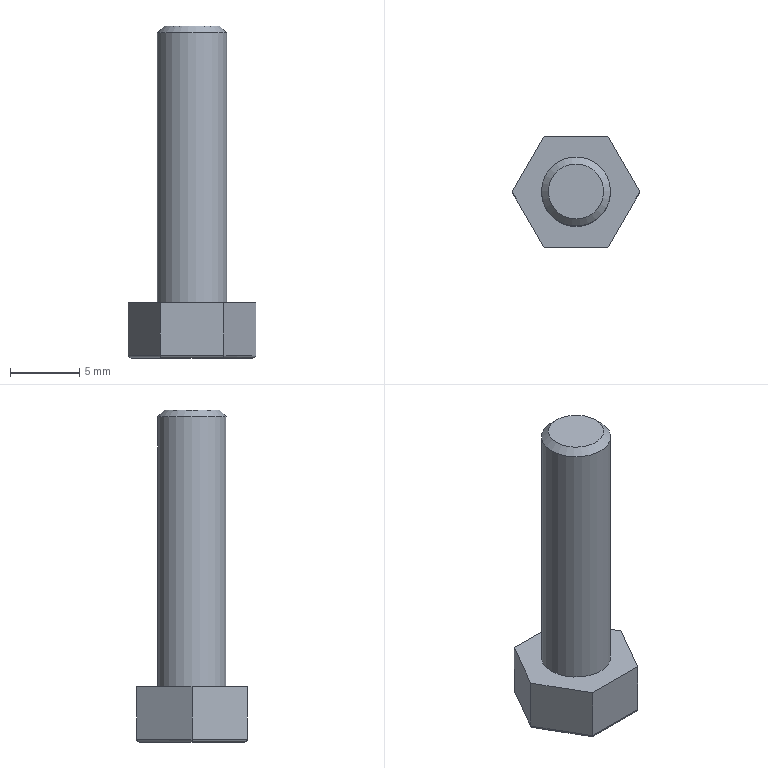Component | NX | BOLT_4 | 1 solid | 17 faces | box 9.24 x 8 x 24 mm | volume 612 mm3 | plane 9 | cylinder 7 | cone 1 | commonest cylinder face diameters 0.4 x6 5 x1
STEP:
#1=CARTESIAN_POINT('',(0.,0.,0.));
#2=DIRECTION('',(0.,0.,1.));
#3=DIRECTION('',(1.,0.,0.));
#4=AXIS2_PLACEMENT_3D('',#1,#2,#3);
#5=CARTESIAN_POINT('',(22.453,0.,12.));
#6=VERTEX_POINT('',#5);
#7=CARTESIAN_POINT('',(20.453,0.,12.));
#8=DIRECTION('',(0.,0.,1.));
#9=DIRECTION('',(1.,0.,0.));
#10=AXIS2_PLACEMENT_3D('',#7,#8,#9);
#11=CIRCLE('',#10,2.);
#12=CARTESIAN_POINT('',(20.453,0.,12.));
#13=DIRECTION('',(0.,0.,1.));
#14=DIRECTION('',(1.,0.,0.));
#15=AXIS2_PLACEMENT_3D('',#12,#13,#14);
#16=PLANE('',#15);
#17=CARTESIAN_POINT('',(0.,0.));
#18=DIRECTION('',(1.,0.));
#19=AXIS2_PLACEMENT_2D('',#17,#18);
#20=CIRCLE('',#19,2.);
#21=(GEOMETRIC_REPRESENTATION_CONTEXT(2)PARAMETRIC_REPRESENTATION_CONTEXT()REPRESENTATION_CONTEXT('',''));
#22=DEFINITIONAL_REPRESENTATION('',(#20),#21);
#23=PCURVE('',#16,#22);
#24=CARTESIAN_POINT('',(20.453,0.,11.5));
#25=DIRECTION('',(0.,0.,-1.));
#26=DIRECTION('',(-1.,0.,0.));
#27=AXIS2_PLACEMENT_3D('',#24,#25,#26);
#28=CONICAL_SURFACE('',#27,2.5,0.7854);
#29=CARTESIAN_POINT('',(9.425,-0.5));
#30=DIRECTION('',(-1.,0.));
#31=VECTOR('',#30,1.);
#32=LINE('',#29,#31);
#33=(GEOMETRIC_REPRESENTATION_CONTEXT(2)PARAMETRIC_REPRESENTATION_CONTEXT()REPRESENTATION_CONTEXT('',''));
#34=DEFINITIONAL_REPRESENTATION('',(#32),#33);
#35=PCURVE('',#28,#34);
#36=SURFACE_CURVE('',#11,(#23,#35),.PCURVE_S1.);
#37=EDGE_CURVE('',#6,#6,#36,.T.);
#38=ORIENTED_EDGE('',*,*,#37,.T.);
#39=EDGE_LOOP('',(#38));
#40=FACE_BOUND('',#39,.T.);
#41=ADVANCED_FACE('',(#40),#16,.T.);
#42=CARTESIAN_POINT('',(22.953,0.,11.5));
#43=VERTEX_POINT('',#42);
#44=CARTESIAN_POINT('',(17.953,-0.,11.5));
#45=VERTEX_POINT('',#44);
#46=CARTESIAN_POINT('',(20.453,0.,11.5));
#47=DIRECTION('',(0.,0.,-1.));
#48=DIRECTION('',(1.,0.,0.));
#49=AXIS2_PLACEMENT_3D('',#46,#47,#48);
#50=CIRCLE('',#49,2.5);
#51=CARTESIAN_POINT('',(20.453,0.,12.));
#52=DIRECTION('',(0.,0.,-1.));
#53=DIRECTION('',(-1.,0.,0.));
#54=AXIS2_PLACEMENT_3D('',#51,#52,#53);
#55=CYLINDRICAL_SURFACE('',#54,2.5);
#56=CARTESIAN_POINT('',(3.142,0.5));
#57=DIRECTION('',(1.,0.));
#58=VECTOR('',#57,1.);
#59=LINE('',#56,#58);
#60=(GEOMETRIC_REPRESENTATION_CONTEXT(2)PARAMETRIC_REPRESENTATION_CONTEXT()REPRESENTATION_CONTEXT('',''));
#61=DEFINITIONAL_REPRESENTATION('',(#59),#60);
#62=PCURVE('',#55,#61);
#63=CARTESIAN_POINT('',(3.142,0.));
#64=DIRECTION('',(1.,0.));
#65=VECTOR('',#64,1.);
#66=LINE('',#63,#65);
#67=(GEOMETRIC_REPRESENTATION_CONTEXT(2)PARAMETRIC_REPRESENTATION_CONTEXT()REPRESENTATION_CONTEXT('',''));
#68=DEFINITIONAL_REPRESENTATION('',(#66),#67);
#69=PCURVE('',#28,#68);
#70=SURFACE_CURVE('',#50,(#62,#69),.PCURVE_S1.);
#71=EDGE_CURVE('',#43,#45,#70,.T.);
#72=ORIENTED_EDGE('',*,*,#71,.T.);
#73=CARTESIAN_POINT('',(17.953,0.,-8.));
#74=VERTEX_POINT('',#73);
#75=CARTESIAN_POINT('',(17.953,0.,11.5));
#76=CARTESIAN_POINT('',(17.953,0.,-8.));
#77=B_SPLINE_CURVE_WITH_KNOTS('',1,(#75,#76),.UNSPECIFIED.,.F.,.F.,(2,2),(0.5,20.),.PIECEWISE_BEZIER_KNOTS.);
#78=CARTESIAN_POINT('',(6.283,0.));
#79=DIRECTION('',(0.,1.));
#80=VECTOR('',#79,1.);
#81=LINE('',#78,#80);
#82=(GEOMETRIC_REPRESENTATION_CONTEXT(2)PARAMETRIC_REPRESENTATION_CONTEXT()REPRESENTATION_CONTEXT('',''));
#83=DEFINITIONAL_REPRESENTATION('',(#81),#82);
#84=PCURVE('',#55,#83);
#85=CARTESIAN_POINT('',(0.,0.));
#86=DIRECTION('',(0.,1.));
#87=VECTOR('',#86,1.);
#88=LINE('',#85,#87);
#89=(GEOMETRIC_REPRESENTATION_CONTEXT(2)PARAMETRIC_REPRESENTATION_CONTEXT()REPRESENTATION_CONTEXT('',''));
#90=DEFINITIONAL_REPRESENTATION('',(#88),#89);
#91=PCURVE('',#55,#90);
#92=SEAM_CURVE('',#77,(#84,#91),.PCURVE_S1.);
#93=EDGE_CURVE('',#45,#74,#92,.T.);
#94=ORIENTED_EDGE('',*,*,#93,.T.);
#95=CARTESIAN_POINT('',(20.453,0.,-8.));
#96=DIRECTION('',(0.,0.,1.));
#97=DIRECTION('',(-1.,0.,0.));
#98=AXIS2_PLACEMENT_3D('',#95,#96,#97);
#99=CIRCLE('',#98,2.5);
#100=CARTESIAN_POINT('',(6.283,20.));
#101=DIRECTION('',(-1.,0.));
#102=VECTOR('',#101,1.);
#103=LINE('',#100,#102);
#104=(GEOMETRIC_REPRESENTATION_CONTEXT(2)PARAMETRIC_REPRESENTATION_CONTEXT()REPRESENTATION_CONTEXT('',''));
#105=DEFINITIONAL_REPRESENTATION('',(#103),#104);
#106=PCURVE('',#55,#105);
#107=CARTESIAN_POINT('',(20.453,0.,-8.));
#108=DIRECTION('',(0.,0.,-1.));
#109=DIRECTION('',(-1.,0.,0.));
#110=AXIS2_PLACEMENT_3D('',#107,#108,#109);
#111=PLANE('',#110);
#112=CARTESIAN_POINT('',(2.5,0.));
#113=CARTESIAN_POINT('',(2.5,-4.33));
#114=CARTESIAN_POINT('',(-1.25,-2.165));
#115=CARTESIAN_POINT('',(-5.,-0.));
#116=CARTESIAN_POINT('',(-1.25,2.165));
#117=CARTESIAN_POINT('',(2.5,4.33));
#118=CARTESIAN_POINT('',(2.5,0.));
#119=(BOUNDED_CURVE()B_SPLINE_CURVE(2,(#112,#113,#114,#115,#116,#117,#118),.UNSPECIFIED.,.T.,.F.)B_SPLINE_CURVE_WITH_KNOTS((1,2,2,2,2,1),(-2.094,0.,2.094,4.189,6.283,8.378),.UNSPECIFIED.)CURVE()GEOMETRIC_REPRESENTATION_ITEM()RATIONAL_B_SPLINE_CURVE((1.,0.5,1.,0.5,1.,0.5,1.))REPRESENTATION_ITEM(''));
#120=(GEOMETRIC_REPRESENTATION_CONTEXT(2)PARAMETRIC_REPRESENTATION_CONTEXT()REPRESENTATION_CONTEXT('',''));
#121=DEFINITIONAL_REPRESENTATION('',(#119),#120);
#122=PCURVE('',#111,#121);
#123=SURFACE_CURVE('',#99,(#106,#122),.PCURVE_S1.);
#124=EDGE_CURVE('',#74,#74,#123,.T.);
#125=ORIENTED_EDGE('',*,*,#124,.T.);
#126=ORIENTED_EDGE('',*,*,#93,.F.);
#127=CARTESIAN_POINT('',(20.453,0.,11.5));
#128=DIRECTION('',(0.,0.,-1.));
#129=DIRECTION('',(1.,0.,0.));
#130=AXIS2_PLACEMENT_3D('',#127,#128,#129);
#131=CIRCLE('',#130,2.5);
#132=CARTESIAN_POINT('',(-3.142,0.5));
#133=DIRECTION('',(1.,0.));
#134=VECTOR('',#133,1.);
#135=LINE('',#132,#134);
#136=(GEOMETRIC_REPRESENTATION_CONTEXT(2)PARAMETRIC_REPRESENTATION_CONTEXT()REPRESENTATION_CONTEXT('',''));
#137=DEFINITIONAL_REPRESENTATION('',(#135),#136);
#138=PCURVE('',#55,#137);
#139=CARTESIAN_POINT('',(3.142,0.));
#140=DIRECTION('',(1.,0.));
#141=VECTOR('',#140,1.);
#142=LINE('',#139,#141);
#143=(GEOMETRIC_REPRESENTATION_CONTEXT(2)PARAMETRIC_REPRESENTATION_CONTEXT()REPRESENTATION_CONTEXT('',''));
#144=DEFINITIONAL_REPRESENTATION('',(#142),#143);
#145=PCURVE('',#28,#144);
#146=SURFACE_CURVE('',#131,(#138,#145),.PCURVE_S1.);
#147=EDGE_CURVE('',#45,#43,#146,.T.);
#148=ORIENTED_EDGE('',*,*,#147,.T.);
#149=EDGE_LOOP('',(#72,#94,#125,#126,#148));
#150=FACE_BOUND('',#149,.T.);
#151=ADVANCED_FACE('',(#150),#55,.T.);
#152=CARTESIAN_POINT('',(18.143,4.,-11.8));
#153=VERTEX_POINT('',#152);
#154=CARTESIAN_POINT('',(18.143,4.,-8.));
#155=VERTEX_POINT('',#154);
#156=CARTESIAN_POINT('',(18.143,4.,-12.));
#157=DIRECTION('',(0.,0.,1.));
#158=VECTOR('',#157,1.);
#159=LINE('',#156,#158);
#160=CARTESIAN_POINT('',(15.834,-0.,-12.));
#161=DIRECTION('',(0.866,-0.5,0.));
#162=DIRECTION('',(-0.5,-0.866,0.));
#163=AXIS2_PLACEMENT_3D('',#160,#161,#162);
#164=PLANE('',#163);
#165=CARTESIAN_POINT('',(-4.619,0.));
#166=DIRECTION('',(0.,-1.));
#167=VECTOR('',#166,1.);
#168=LINE('',#165,#167);
#169=(GEOMETRIC_REPRESENTATION_CONTEXT(2)PARAMETRIC_REPRESENTATION_CONTEXT()REPRESENTATION_CONTEXT('',''));
#170=DEFINITIONAL_REPRESENTATION('',(#168),#169);
#171=PCURVE('',#164,#170);
#172=CARTESIAN_POINT('',(18.143,4.,-12.));
#173=DIRECTION('',(0.,-1.,0.));
#174=DIRECTION('',(0.,0.,1.));
#175=AXIS2_PLACEMENT_3D('',#172,#173,#174);
#176=PLANE('',#175);
#177=CARTESIAN_POINT('',(0.,0.));
#178=DIRECTION('',(1.,0.));
#179=VECTOR('',#178,1.);
#180=LINE('',#177,#179);
#181=(GEOMETRIC_REPRESENTATION_CONTEXT(2)PARAMETRIC_REPRESENTATION_CONTEXT()REPRESENTATION_CONTEXT('',''));
#182=DEFINITIONAL_REPRESENTATION('',(#180),#181);
#183=PCURVE('',#176,#182);
#184=SURFACE_CURVE('',#159,(#171,#183),.PCURVE_S1.);
#185=EDGE_CURVE('',#153,#155,#184,.T.);
#186=ORIENTED_EDGE('',*,*,#185,.F.);
#187=CARTESIAN_POINT('',(15.834,-0.,-11.8));
#188=VERTEX_POINT('',#187);
#189=CARTESIAN_POINT('',(15.834,-0.,-11.8));
#190=DIRECTION('',(-0.5,-0.866,0.));
#191=VECTOR('',#190,1.);
#192=LINE('',#189,#191);
#193=CARTESIAN_POINT('',(0.,-0.2));
#194=DIRECTION('',(1.,0.));
#195=VECTOR('',#194,1.);
#196=LINE('',#193,#195);
#197=(GEOMETRIC_REPRESENTATION_CONTEXT(2)PARAMETRIC_REPRESENTATION_CONTEXT()REPRESENTATION_CONTEXT('',''));
#198=DEFINITIONAL_REPRESENTATION('',(#196),#197);
#199=PCURVE('',#164,#198);
#200=CARTESIAN_POINT('',(17.162,1.9,-11.8));
#201=DIRECTION('',(-0.5,-0.866,0.));
#202=DIRECTION('',(-0.866,0.5,0.));
#203=AXIS2_PLACEMENT_3D('',#200,#201,#202);
#204=CYLINDRICAL_SURFACE('',#203,0.2);
#205=CARTESIAN_POINT('',(0.,2.309));
#206=DIRECTION('',(0.,1.));
#207=VECTOR('',#206,1.);
#208=LINE('',#205,#207);
#209=(GEOMETRIC_REPRESENTATION_CONTEXT(2)PARAMETRIC_REPRESENTATION_CONTEXT()REPRESENTATION_CONTEXT('',''));
#210=DEFINITIONAL_REPRESENTATION('',(#208),#209);
#211=PCURVE('',#204,#210);
#212=SURFACE_CURVE('',#192,(#199,#211),.PCURVE_S1.);
#213=EDGE_CURVE('',#153,#188,#212,.T.);
#214=ORIENTED_EDGE('',*,*,#213,.T.);
#215=CARTESIAN_POINT('',(15.834,-0.,-8.));
#216=VERTEX_POINT('',#215);
#217=CARTESIAN_POINT('',(15.834,-0.,-12.));
#218=DIRECTION('',(0.,0.,1.));
#219=VECTOR('',#218,1.);
#220=LINE('',#217,#219);
#221=CARTESIAN_POINT('',(0.,0.));
#222=DIRECTION('',(0.,-1.));
#223=VECTOR('',#222,1.);
#224=LINE('',#221,#223);
#225=(GEOMETRIC_REPRESENTATION_CONTEXT(2)PARAMETRIC_REPRESENTATION_CONTEXT()REPRESENTATION_CONTEXT('',''));
#226=DEFINITIONAL_REPRESENTATION('',(#224),#225);
#227=PCURVE('',#164,#226);
#228=CARTESIAN_POINT('',(18.143,-4.,-12.));
#229=DIRECTION('',(0.866,0.5,0.));
#230=DIRECTION('',(0.5,-0.866,0.));
#231=AXIS2_PLACEMENT_3D('',#228,#229,#230);
#232=PLANE('',#231);
#233=CARTESIAN_POINT('',(-4.619,0.));
#234=DIRECTION('',(0.,-1.));
#235=VECTOR('',#234,1.);
#236=LINE('',#233,#235);
#237=(GEOMETRIC_REPRESENTATION_CONTEXT(2)PARAMETRIC_REPRESENTATION_CONTEXT()REPRESENTATION_CONTEXT('',''));
#238=DEFINITIONAL_REPRESENTATION('',(#236),#237);
#239=PCURVE('',#232,#238);
#240=SURFACE_CURVE('',#220,(#227,#239),.PCURVE_S1.);
#241=EDGE_CURVE('',#188,#216,#240,.T.);
#242=ORIENTED_EDGE('',*,*,#241,.T.);
#243=CARTESIAN_POINT('',(15.834,-0.,-8.));
#244=DIRECTION('',(0.5,0.866,0.));
#245=VECTOR('',#244,1.);
#246=LINE('',#243,#245);
#247=CARTESIAN_POINT('',(0.,-4.));
#248=DIRECTION('',(-1.,0.));
#249=VECTOR('',#248,1.);
#250=LINE('',#247,#249);
#251=(GEOMETRIC_REPRESENTATION_CONTEXT(2)PARAMETRIC_REPRESENTATION_CONTEXT()REPRESENTATION_CONTEXT('',''));
#252=DEFINITIONAL_REPRESENTATION('',(#250),#251);
#253=PCURVE('',#164,#252);
#254=CARTESIAN_POINT('',(4.619,-0.));
#255=DIRECTION('',(-0.5,0.866));
#256=VECTOR('',#255,1.);
#257=LINE('',#254,#256);
#258=(GEOMETRIC_REPRESENTATION_CONTEXT(2)PARAMETRIC_REPRESENTATION_CONTEXT()REPRESENTATION_CONTEXT('',''));
#259=DEFINITIONAL_REPRESENTATION('',(#257),#258);
#260=PCURVE('',#111,#259);
#261=SURFACE_CURVE('',#246,(#253,#260),.PCURVE_S1.);
#262=EDGE_CURVE('',#216,#155,#261,.T.);
#263=ORIENTED_EDGE('',*,*,#262,.T.);
#264=EDGE_LOOP('',(#186,#214,#242,#263));
#265=FACE_BOUND('',#264,.T.);
#266=ADVANCED_FACE('',(#265),#164,.F.);
#267=CARTESIAN_POINT('',(22.762,4.,-11.8));
#268=VERTEX_POINT('',#267);
#269=CARTESIAN_POINT('',(22.762,4.,-8.));
#270=VERTEX_POINT('',#269);
#271=CARTESIAN_POINT('',(22.762,4.,-12.));
#272=DIRECTION('',(0.,0.,1.));
#273=VECTOR('',#272,1.);
#274=LINE('',#271,#273);
#275=CARTESIAN_POINT('',(0.,-4.619));
#276=DIRECTION('',(1.,0.));
#277=VECTOR('',#276,1.);
#278=LINE('',#275,#277);
#279=(GEOMETRIC_REPRESENTATION_CONTEXT(2)PARAMETRIC_REPRESENTATION_CONTEXT()REPRESENTATION_CONTEXT('',''));
#280=DEFINITIONAL_REPRESENTATION('',(#278),#279);
#281=PCURVE('',#176,#280);
#282=CARTESIAN_POINT('',(22.762,4.,-12.));
#283=DIRECTION('',(-0.866,-0.5,0.));
#284=DIRECTION('',(-0.5,0.866,0.));
#285=AXIS2_PLACEMENT_3D('',#282,#283,#284);
#286=PLANE('',#285);
#287=CARTESIAN_POINT('',(0.,0.));
#288=DIRECTION('',(0.,-1.));
#289=VECTOR('',#288,1.);
#290=LINE('',#287,#289);
#291=(GEOMETRIC_REPRESENTATION_CONTEXT(2)PARAMETRIC_REPRESENTATION_CONTEXT()REPRESENTATION_CONTEXT('',''));
#292=DEFINITIONAL_REPRESENTATION('',(#290),#291);
#293=PCURVE('',#286,#292);
#294=SURFACE_CURVE('',#274,(#281,#293),.PCURVE_S1.);
#295=EDGE_CURVE('',#268,#270,#294,.T.);
#296=ORIENTED_EDGE('',*,*,#295,.F.);
#297=CARTESIAN_POINT('',(18.143,4.,-11.8));
#298=DIRECTION('',(-1.,0.,0.));
#299=VECTOR('',#298,1.);
#300=LINE('',#297,#299);
#301=CARTESIAN_POINT('',(0.2,0.));
#302=DIRECTION('',(0.,1.));
#303=VECTOR('',#302,1.);
#304=LINE('',#301,#303);
#305=(GEOMETRIC_REPRESENTATION_CONTEXT(2)PARAMETRIC_REPRESENTATION_CONTEXT()REPRESENTATION_CONTEXT('',''));
#306=DEFINITIONAL_REPRESENTATION('',(#304),#305);
#307=PCURVE('',#176,#306);
#308=CARTESIAN_POINT('',(20.453,3.8,-11.8));
#309=DIRECTION('',(-1.,0.,0.));
#310=DIRECTION('',(0.,0.,1.));
#311=AXIS2_PLACEMENT_3D('',#308,#309,#310);
#312=CYLINDRICAL_SURFACE('',#311,0.2);
#313=CARTESIAN_POINT('',(1.571,2.309));
#314=DIRECTION('',(0.,1.));
#315=VECTOR('',#314,1.);
#316=LINE('',#313,#315);
#317=(GEOMETRIC_REPRESENTATION_CONTEXT(2)PARAMETRIC_REPRESENTATION_CONTEXT()REPRESENTATION_CONTEXT('',''));
#318=DEFINITIONAL_REPRESENTATION('',(#316),#317);
#319=PCURVE('',#312,#318);
#320=SURFACE_CURVE('',#300,(#307,#319),.PCURVE_S1.);
#321=EDGE_CURVE('',#268,#153,#320,.T.);
#322=ORIENTED_EDGE('',*,*,#321,.T.);
#323=ORIENTED_EDGE('',*,*,#185,.T.);
#324=CARTESIAN_POINT('',(18.143,4.,-8.));
#325=DIRECTION('',(1.,0.,0.));
#326=VECTOR('',#325,1.);
#327=LINE('',#324,#326);
#328=CARTESIAN_POINT('',(4.,0.));
#329=DIRECTION('',(0.,-1.));
#330=VECTOR('',#329,1.);
#331=LINE('',#328,#330);
#332=(GEOMETRIC_REPRESENTATION_CONTEXT(2)PARAMETRIC_REPRESENTATION_CONTEXT()REPRESENTATION_CONTEXT('',''));
#333=DEFINITIONAL_REPRESENTATION('',(#331),#332);
#334=PCURVE('',#176,#333);
#335=CARTESIAN_POINT('',(2.309,4.));
#336=DIRECTION('',(-1.,0.));
#337=VECTOR('',#336,1.);
#338=LINE('',#335,#337);
#339=(GEOMETRIC_REPRESENTATION_CONTEXT(2)PARAMETRIC_REPRESENTATION_CONTEXT()REPRESENTATION_CONTEXT('',''));
#340=DEFINITIONAL_REPRESENTATION('',(#338),#339);
#341=PCURVE('',#111,#340);
#342=SURFACE_CURVE('',#327,(#334,#341),.PCURVE_S1.);
#343=EDGE_CURVE('',#155,#270,#342,.T.);
#344=ORIENTED_EDGE('',*,*,#343,.T.);
#345=EDGE_LOOP('',(#296,#322,#323,#344));
#346=FACE_BOUND('',#345,.T.);
#347=ADVANCED_FACE('',(#346),#176,.F.);
#348=CARTESIAN_POINT('',(25.072,0.,-11.8));
#349=VERTEX_POINT('',#348);
#350=CARTESIAN_POINT('',(25.072,0.,-8.));
#351=VERTEX_POINT('',#350);
#352=CARTESIAN_POINT('',(25.072,0.,-12.));
#353=DIRECTION('',(0.,0.,1.));
#354=VECTOR('',#353,1.);
#355=LINE('',#352,#354);
#356=CARTESIAN_POINT('',(-4.619,0.));
#357=DIRECTION('',(0.,-1.));
#358=VECTOR('',#357,1.);
#359=LINE('',#356,#358);
#360=(GEOMETRIC_REPRESENTATION_CONTEXT(2)PARAMETRIC_REPRESENTATION_CONTEXT()REPRESENTATION_CONTEXT('',''));
#361=DEFINITIONAL_REPRESENTATION('',(#359),#360);
#362=PCURVE('',#286,#361);
#363=CARTESIAN_POINT('',(25.072,0.,-12.));
#364=DIRECTION('',(-0.866,0.5,0.));
#365=DIRECTION('',(0.5,0.866,0.));
#366=AXIS2_PLACEMENT_3D('',#363,#364,#365);
#367=PLANE('',#366);
#368=CARTESIAN_POINT('',(0.,0.));
#369=DIRECTION('',(0.,-1.));
#370=VECTOR('',#369,1.);
#371=LINE('',#368,#370);
#372=(GEOMETRIC_REPRESENTATION_CONTEXT(2)PARAMETRIC_REPRESENTATION_CONTEXT()REPRESENTATION_CONTEXT('',''));
#373=DEFINITIONAL_REPRESENTATION('',(#371),#372);
#374=PCURVE('',#367,#373);
#375=SURFACE_CURVE('',#355,(#362,#374),.PCURVE_S1.);
#376=EDGE_CURVE('',#349,#351,#375,.T.);
#377=ORIENTED_EDGE('',*,*,#376,.F.);
#378=CARTESIAN_POINT('',(22.762,4.,-11.8));
#379=DIRECTION('',(-0.5,0.866,0.));
#380=VECTOR('',#379,1.);
#381=LINE('',#378,#380);
#382=CARTESIAN_POINT('',(0.,-0.2));
#383=DIRECTION('',(1.,0.));
#384=VECTOR('',#383,1.);
#385=LINE('',#382,#384);
#386=(GEOMETRIC_REPRESENTATION_CONTEXT(2)PARAMETRIC_REPRESENTATION_CONTEXT()REPRESENTATION_CONTEXT('',''));
#387=DEFINITIONAL_REPRESENTATION('',(#385),#386);
#388=PCURVE('',#286,#387);
#389=CARTESIAN_POINT('',(23.744,1.9,-11.8));
#390=DIRECTION('',(-0.5,0.866,0.));
#391=DIRECTION('',(0.866,0.5,0.));
#392=AXIS2_PLACEMENT_3D('',#389,#390,#391);
#393=CYLINDRICAL_SURFACE('',#392,0.2);
#394=CARTESIAN_POINT('',(0.,2.309));
#395=DIRECTION('',(0.,1.));
#396=VECTOR('',#395,1.);
#397=LINE('',#394,#396);
#398=(GEOMETRIC_REPRESENTATION_CONTEXT(2)PARAMETRIC_REPRESENTATION_CONTEXT()REPRESENTATION_CONTEXT('',''));
#399=DEFINITIONAL_REPRESENTATION('',(#397),#398);
#400=PCURVE('',#393,#399);
#401=SURFACE_CURVE('',#381,(#388,#400),.PCURVE_S1.);
#402=EDGE_CURVE('',#349,#268,#401,.T.);
#403=ORIENTED_EDGE('',*,*,#402,.T.);
#404=ORIENTED_EDGE('',*,*,#295,.T.);
#405=CARTESIAN_POINT('',(22.762,4.,-8.));
#406=DIRECTION('',(0.5,-0.866,0.));
#407=VECTOR('',#406,1.);
#408=LINE('',#405,#407);
#409=CARTESIAN_POINT('',(0.,-4.));
#410=DIRECTION('',(-1.,0.));
#411=VECTOR('',#410,1.);
#412=LINE('',#409,#411);
#413=(GEOMETRIC_REPRESENTATION_CONTEXT(2)PARAMETRIC_REPRESENTATION_CONTEXT()REPRESENTATION_CONTEXT('',''));
#414=DEFINITIONAL_REPRESENTATION('',(#412),#413);
#415=PCURVE('',#286,#414);
#416=CARTESIAN_POINT('',(-2.309,4.));
#417=DIRECTION('',(-0.5,-0.866));
#418=VECTOR('',#417,1.);
#419=LINE('',#416,#418);
#420=(GEOMETRIC_REPRESENTATION_CONTEXT(2)PARAMETRIC_REPRESENTATION_CONTEXT()REPRESENTATION_CONTEXT('',''));
#421=DEFINITIONAL_REPRESENTATION('',(#419),#420);
#422=PCURVE('',#111,#421);
#423=SURFACE_CURVE('',#408,(#415,#422),.PCURVE_S1.);
#424=EDGE_CURVE('',#270,#351,#423,.T.);
#425=ORIENTED_EDGE('',*,*,#424,.T.);
#426=EDGE_LOOP('',(#377,#403,#404,#425));
#427=FACE_BOUND('',#426,.T.);
#428=ADVANCED_FACE('',(#427),#286,.F.);
#429=CARTESIAN_POINT('',(22.762,-4.,-11.8));
#430=VERTEX_POINT('',#429);
#431=CARTESIAN_POINT('',(22.762,-4.,-8.));
#432=VERTEX_POINT('',#431);
#433=CARTESIAN_POINT('',(22.762,-4.,-12.));
#434=DIRECTION('',(0.,0.,1.));
#435=VECTOR('',#434,1.);
#436=LINE('',#433,#435);
#437=CARTESIAN_POINT('',(-4.619,0.));
#438=DIRECTION('',(0.,-1.));
#439=VECTOR('',#438,1.);
#440=LINE('',#437,#439);
#441=(GEOMETRIC_REPRESENTATION_CONTEXT(2)PARAMETRIC_REPRESENTATION_CONTEXT()REPRESENTATION_CONTEXT('',''));
#442=DEFINITIONAL_REPRESENTATION('',(#440),#441);
#443=PCURVE('',#367,#442);
#444=CARTESIAN_POINT('',(22.762,-4.,-12.));
#445=DIRECTION('',(0.,1.,0.));
#446=DIRECTION('',(0.,0.,-1.));
#447=AXIS2_PLACEMENT_3D('',#444,#445,#446);
#448=PLANE('',#447);
#449=CARTESIAN_POINT('',(0.,0.));
#450=DIRECTION('',(-1.,0.));
#451=VECTOR('',#450,1.);
#452=LINE('',#449,#451);
#453=(GEOMETRIC_REPRESENTATION_CONTEXT(2)PARAMETRIC_REPRESENTATION_CONTEXT()REPRESENTATION_CONTEXT('',''));
#454=DEFINITIONAL_REPRESENTATION('',(#452),#453);
#455=PCURVE('',#448,#454);
#456=SURFACE_CURVE('',#436,(#443,#455),.PCURVE_S1.);
#457=EDGE_CURVE('',#430,#432,#456,.T.);
#458=ORIENTED_EDGE('',*,*,#457,.F.);
#459=CARTESIAN_POINT('',(25.072,0.,-11.8));
#460=DIRECTION('',(0.5,0.866,0.));
#461=VECTOR('',#460,1.);
#462=LINE('',#459,#461);
#463=CARTESIAN_POINT('',(0.,-0.2));
#464=DIRECTION('',(1.,0.));
#465=VECTOR('',#464,1.);
#466=LINE('',#463,#465);
#467=(GEOMETRIC_REPRESENTATION_CONTEXT(2)PARAMETRIC_REPRESENTATION_CONTEXT()REPRESENTATION_CONTEXT('',''));
#468=DEFINITIONAL_REPRESENTATION('',(#466),#467);
#469=PCURVE('',#367,#468);
#470=CARTESIAN_POINT('',(23.744,-1.9,-11.8));
#471=DIRECTION('',(0.5,0.866,0.));
#472=DIRECTION('',(0.866,-0.5,0.));
#473=AXIS2_PLACEMENT_3D('',#470,#471,#472);
#474=CYLINDRICAL_SURFACE('',#473,0.2);
#475=CARTESIAN_POINT('',(0.,2.309));
#476=DIRECTION('',(0.,1.));
#477=VECTOR('',#476,1.);
#478=LINE('',#475,#477);
#479=(GEOMETRIC_REPRESENTATION_CONTEXT(2)PARAMETRIC_REPRESENTATION_CONTEXT()REPRESENTATION_CONTEXT('',''));
#480=DEFINITIONAL_REPRESENTATION('',(#478),#479);
#481=PCURVE('',#474,#480);
#482=SURFACE_CURVE('',#462,(#469,#481),.PCURVE_S1.);
#483=EDGE_CURVE('',#430,#349,#482,.T.);
#484=ORIENTED_EDGE('',*,*,#483,.T.);
#485=ORIENTED_EDGE('',*,*,#376,.T.);
#486=CARTESIAN_POINT('',(25.072,0.,-8.));
#487=DIRECTION('',(-0.5,-0.866,0.));
#488=VECTOR('',#487,1.);
#489=LINE('',#486,#488);
#490=CARTESIAN_POINT('',(0.,-4.));
#491=DIRECTION('',(-1.,0.));
#492=VECTOR('',#491,1.);
#493=LINE('',#490,#492);
#494=(GEOMETRIC_REPRESENTATION_CONTEXT(2)PARAMETRIC_REPRESENTATION_CONTEXT()REPRESENTATION_CONTEXT('',''));
#495=DEFINITIONAL_REPRESENTATION('',(#493),#494);
#496=PCURVE('',#367,#495);
#497=CARTESIAN_POINT('',(-4.619,0.));
#498=DIRECTION('',(0.5,-0.866));
#499=VECTOR('',#498,1.);
#500=LINE('',#497,#499);
#501=(GEOMETRIC_REPRESENTATION_CONTEXT(2)PARAMETRIC_REPRESENTATION_CONTEXT()REPRESENTATION_CONTEXT('',''));
#502=DEFINITIONAL_REPRESENTATION('',(#500),#501);
#503=PCURVE('',#111,#502);
#504=SURFACE_CURVE('',#489,(#496,#503),.PCURVE_S1.);
#505=EDGE_CURVE('',#351,#432,#504,.T.);
#506=ORIENTED_EDGE('',*,*,#505,.T.);
#507=EDGE_LOOP('',(#458,#484,#485,#506));
#508=FACE_BOUND('',#507,.T.);
#509=ADVANCED_FACE('',(#508),#367,.F.);
#510=CARTESIAN_POINT('',(18.143,-4.,-11.8));
#511=VERTEX_POINT('',#510);
#512=CARTESIAN_POINT('',(18.143,-4.,-8.));
#513=VERTEX_POINT('',#512);
#514=CARTESIAN_POINT('',(18.143,-4.,-12.));
#515=DIRECTION('',(0.,0.,1.));
#516=VECTOR('',#515,1.);
#517=LINE('',#514,#516);
#518=CARTESIAN_POINT('',(0.,4.619));
#519=DIRECTION('',(-1.,0.));
#520=VECTOR('',#519,1.);
#521=LINE('',#518,#520);
#522=(GEOMETRIC_REPRESENTATION_CONTEXT(2)PARAMETRIC_REPRESENTATION_CONTEXT()REPRESENTATION_CONTEXT('',''));
#523=DEFINITIONAL_REPRESENTATION('',(#521),#522);
#524=PCURVE('',#448,#523);
#525=CARTESIAN_POINT('',(0.,0.));
#526=DIRECTION('',(0.,-1.));
#527=VECTOR('',#526,1.);
#528=LINE('',#525,#527);
#529=(GEOMETRIC_REPRESENTATION_CONTEXT(2)PARAMETRIC_REPRESENTATION_CONTEXT()REPRESENTATION_CONTEXT('',''));
#530=DEFINITIONAL_REPRESENTATION('',(#528),#529);
#531=PCURVE('',#232,#530);
#532=SURFACE_CURVE('',#517,(#524,#531),.PCURVE_S1.);
#533=EDGE_CURVE('',#511,#513,#532,.T.);
#534=ORIENTED_EDGE('',*,*,#533,.F.);
#535=CARTESIAN_POINT('',(22.762,-4.,-11.8));
#536=DIRECTION('',(1.,0.,0.));
#537=VECTOR('',#536,1.);
#538=LINE('',#535,#537);
#539=CARTESIAN_POINT('',(-0.2,0.));
#540=DIRECTION('',(0.,-1.));
#541=VECTOR('',#540,1.);
#542=LINE('',#539,#541);
#543=(GEOMETRIC_REPRESENTATION_CONTEXT(2)PARAMETRIC_REPRESENTATION_CONTEXT()REPRESENTATION_CONTEXT('',''));
#544=DEFINITIONAL_REPRESENTATION('',(#542),#543);
#545=PCURVE('',#448,#544);
#546=CARTESIAN_POINT('',(20.453,-3.8,-11.8));
#547=DIRECTION('',(1.,0.,0.));
#548=DIRECTION('',(0.,0.,-1.));
#549=AXIS2_PLACEMENT_3D('',#546,#547,#548);
#550=CYLINDRICAL_SURFACE('',#549,0.2);
#551=CARTESIAN_POINT('',(4.712,2.309));
#552=DIRECTION('',(0.,1.));
#553=VECTOR('',#552,1.);
#554=LINE('',#551,#553);
#555=(GEOMETRIC_REPRESENTATION_CONTEXT(2)PARAMETRIC_REPRESENTATION_CONTEXT()REPRESENTATION_CONTEXT('',''));
#556=DEFINITIONAL_REPRESENTATION('',(#554),#555);
#557=PCURVE('',#550,#556);
#558=SURFACE_CURVE('',#538,(#545,#557),.PCURVE_S1.);
#559=EDGE_CURVE('',#511,#430,#558,.T.);
#560=ORIENTED_EDGE('',*,*,#559,.T.);
#561=ORIENTED_EDGE('',*,*,#457,.T.);
#562=CARTESIAN_POINT('',(22.762,-4.,-8.));
#563=DIRECTION('',(-1.,0.,0.));
#564=VECTOR('',#563,1.);
#565=LINE('',#562,#564);
#566=CARTESIAN_POINT('',(-4.,0.));
#567=DIRECTION('',(0.,1.));
#568=VECTOR('',#567,1.);
#569=LINE('',#566,#568);
#570=(GEOMETRIC_REPRESENTATION_CONTEXT(2)PARAMETRIC_REPRESENTATION_CONTEXT()REPRESENTATION_CONTEXT('',''));
#571=DEFINITIONAL_REPRESENTATION('',(#569),#570);
#572=PCURVE('',#448,#571);
#573=CARTESIAN_POINT('',(-2.309,-4.));
#574=DIRECTION('',(1.,0.));
#575=VECTOR('',#574,1.);
#576=LINE('',#573,#575);
#577=(GEOMETRIC_REPRESENTATION_CONTEXT(2)PARAMETRIC_REPRESENTATION_CONTEXT()REPRESENTATION_CONTEXT('',''));
#578=DEFINITIONAL_REPRESENTATION('',(#576),#577);
#579=PCURVE('',#111,#578);
#580=SURFACE_CURVE('',#565,(#572,#579),.PCURVE_S1.);
#581=EDGE_CURVE('',#432,#513,#580,.T.);
#582=ORIENTED_EDGE('',*,*,#581,.T.);
#583=EDGE_LOOP('',(#534,#560,#561,#582));
#584=FACE_BOUND('',#583,.T.);
#585=ADVANCED_FACE('',(#584),#448,.F.);
#586=ORIENTED_EDGE('',*,*,#241,.F.);
#587=CARTESIAN_POINT('',(18.143,-4.,-11.8));
#588=DIRECTION('',(0.5,-0.866,0.));
#589=VECTOR('',#588,1.);
#590=LINE('',#587,#589);
#591=CARTESIAN_POINT('',(0.,-0.2));
#592=DIRECTION('',(1.,0.));
#593=VECTOR('',#592,1.);
#594=LINE('',#591,#593);
#595=(GEOMETRIC_REPRESENTATION_CONTEXT(2)PARAMETRIC_REPRESENTATION_CONTEXT()REPRESENTATION_CONTEXT('',''));
#596=DEFINITIONAL_REPRESENTATION('',(#594),#595);
#597=PCURVE('',#232,#596);
#598=CARTESIAN_POINT('',(17.162,-1.9,-11.8));
#599=DIRECTION('',(0.5,-0.866,0.));
#600=DIRECTION('',(-0.866,-0.5,0.));
#601=AXIS2_PLACEMENT_3D('',#598,#599,#600);
#602=CYLINDRICAL_SURFACE('',#601,0.2);
#603=CARTESIAN_POINT('',(0.,2.309));
#604=DIRECTION('',(0.,1.));
#605=VECTOR('',#604,1.);
#606=LINE('',#603,#605);
#607=(GEOMETRIC_REPRESENTATION_CONTEXT(2)PARAMETRIC_REPRESENTATION_CONTEXT()REPRESENTATION_CONTEXT('',''));
#608=DEFINITIONAL_REPRESENTATION('',(#606),#607);
#609=PCURVE('',#602,#608);
#610=SURFACE_CURVE('',#590,(#597,#609),.PCURVE_S1.);
#611=EDGE_CURVE('',#188,#511,#610,.T.);
#612=ORIENTED_EDGE('',*,*,#611,.T.);
#613=ORIENTED_EDGE('',*,*,#533,.T.);
#614=CARTESIAN_POINT('',(18.143,-4.,-8.));
#615=DIRECTION('',(-0.5,0.866,0.));
#616=VECTOR('',#615,1.);
#617=LINE('',#614,#616);
#618=CARTESIAN_POINT('',(0.,-4.));
#619=DIRECTION('',(-1.,0.));
#620=VECTOR('',#619,1.);
#621=LINE('',#618,#620);
#622=(GEOMETRIC_REPRESENTATION_CONTEXT(2)PARAMETRIC_REPRESENTATION_CONTEXT()REPRESENTATION_CONTEXT('',''));
#623=DEFINITIONAL_REPRESENTATION('',(#621),#622);
#624=PCURVE('',#232,#623);
#625=CARTESIAN_POINT('',(2.309,-4.));
#626=DIRECTION('',(0.5,0.866));
#627=VECTOR('',#626,1.);
#628=LINE('',#625,#627);
#629=(GEOMETRIC_REPRESENTATION_CONTEXT(2)PARAMETRIC_REPRESENTATION_CONTEXT()REPRESENTATION_CONTEXT('',''));
#630=DEFINITIONAL_REPRESENTATION('',(#628),#629);
#631=PCURVE('',#111,#630);
#632=SURFACE_CURVE('',#617,(#624,#631),.PCURVE_S1.);
#633=EDGE_CURVE('',#513,#216,#632,.T.);
#634=ORIENTED_EDGE('',*,*,#633,.T.);
#635=EDGE_LOOP('',(#586,#612,#613,#634));
#636=FACE_BOUND('',#635,.T.);
#637=ADVANCED_FACE('',(#636),#232,.F.);
#638=CARTESIAN_POINT('',(22.647,3.8,-12.));
#639=VERTEX_POINT('',#638);
#640=CARTESIAN_POINT('',(24.841,-0.,-12.));
#641=VERTEX_POINT('',#640);
#642=CARTESIAN_POINT('',(24.898,-0.1,-12.));
#643=DIRECTION('',(0.5,-0.866,0.));
#644=VECTOR('',#643,1.);
#645=LINE('',#642,#644);
#646=CARTESIAN_POINT('',(20.453,0.,-12.));
#647=DIRECTION('',(0.,0.,-1.));
#648=DIRECTION('',(-1.,0.,0.));
#649=AXIS2_PLACEMENT_3D('',#646,#647,#648);
#650=PLANE('',#649);
#651=CARTESIAN_POINT('',(-4.446,-0.1));
#652=DIRECTION('',(-0.5,-0.866));
#653=VECTOR('',#652,1.);
#654=LINE('',#651,#653);
#655=(GEOMETRIC_REPRESENTATION_CONTEXT(2)PARAMETRIC_REPRESENTATION_CONTEXT()REPRESENTATION_CONTEXT('',''));
#656=DEFINITIONAL_REPRESENTATION('',(#654),#655);
#657=PCURVE('',#650,#656);
#658=CARTESIAN_POINT('',(1.571,-2.309));
#659=DIRECTION('',(0.,-1.));
#660=VECTOR('',#659,1.);
#661=LINE('',#658,#660);
#662=(GEOMETRIC_REPRESENTATION_CONTEXT(2)PARAMETRIC_REPRESENTATION_CONTEXT()REPRESENTATION_CONTEXT('',''));
#663=DEFINITIONAL_REPRESENTATION('',(#661),#662);
#664=PCURVE('',#393,#663);
#665=SURFACE_CURVE('',#645,(#657,#664),.PCURVE_S1.);
#666=EDGE_CURVE('',#639,#641,#665,.T.);
#667=ORIENTED_EDGE('',*,*,#666,.T.);
#668=CARTESIAN_POINT('',(22.647,-3.8,-12.));
#669=VERTEX_POINT('',#668);
#670=CARTESIAN_POINT('',(22.589,-3.9,-12.));
#671=DIRECTION('',(-0.5,-0.866,0.));
#672=VECTOR('',#671,1.);
#673=LINE('',#670,#672);
#674=CARTESIAN_POINT('',(-2.136,-3.9));
#675=DIRECTION('',(0.5,-0.866));
#676=VECTOR('',#675,1.);
#677=LINE('',#674,#676);
#678=(GEOMETRIC_REPRESENTATION_CONTEXT(2)PARAMETRIC_REPRESENTATION_CONTEXT()REPRESENTATION_CONTEXT('',''));
#679=DEFINITIONAL_REPRESENTATION('',(#677),#678);
#680=PCURVE('',#650,#679);
#681=CARTESIAN_POINT('',(1.571,-2.309));
#682=DIRECTION('',(0.,-1.));
#683=VECTOR('',#682,1.);
#684=LINE('',#681,#683);
#685=(GEOMETRIC_REPRESENTATION_CONTEXT(2)PARAMETRIC_REPRESENTATION_CONTEXT()REPRESENTATION_CONTEXT('',''));
#686=DEFINITIONAL_REPRESENTATION('',(#684),#685);
#687=PCURVE('',#474,#686);
#688=SURFACE_CURVE('',#673,(#680,#687),.PCURVE_S1.);
#689=EDGE_CURVE('',#641,#669,#688,.T.);
#690=ORIENTED_EDGE('',*,*,#689,.T.);
#691=CARTESIAN_POINT('',(18.259,-3.8,-12.));
#692=VERTEX_POINT('',#691);
#693=CARTESIAN_POINT('',(18.143,-3.8,-12.));
#694=DIRECTION('',(-1.,0.,0.));
#695=VECTOR('',#694,1.);
#696=LINE('',#693,#695);
#697=CARTESIAN_POINT('',(2.309,-3.8));
#698=DIRECTION('',(1.,0.));
#699=VECTOR('',#698,1.);
#700=LINE('',#697,#699);
#701=(GEOMETRIC_REPRESENTATION_CONTEXT(2)PARAMETRIC_REPRESENTATION_CONTEXT()REPRESENTATION_CONTEXT('',''));
#702=DEFINITIONAL_REPRESENTATION('',(#700),#701);
#703=PCURVE('',#650,#702);
#704=CARTESIAN_POINT('',(6.283,-2.309));
#705=DIRECTION('',(0.,-1.));
#706=VECTOR('',#705,1.);
#707=LINE('',#704,#706);
#708=(GEOMETRIC_REPRESENTATION_CONTEXT(2)PARAMETRIC_REPRESENTATION_CONTEXT()REPRESENTATION_CONTEXT('',''));
#709=DEFINITIONAL_REPRESENTATION('',(#707),#708);
#710=PCURVE('',#550,#709);
#711=SURFACE_CURVE('',#696,(#703,#710),.PCURVE_S1.);
#712=EDGE_CURVE('',#669,#692,#711,.T.);
#713=ORIENTED_EDGE('',*,*,#712,.T.);
#714=CARTESIAN_POINT('',(16.065,-0.,-12.));
#715=VERTEX_POINT('',#714);
#716=CARTESIAN_POINT('',(16.007,0.1,-12.));
#717=DIRECTION('',(-0.5,0.866,0.));
#718=VECTOR('',#717,1.);
#719=LINE('',#716,#718);
#720=CARTESIAN_POINT('',(4.446,0.1));
#721=DIRECTION('',(0.5,0.866));
#722=VECTOR('',#721,1.);
#723=LINE('',#720,#722);
#724=(GEOMETRIC_REPRESENTATION_CONTEXT(2)PARAMETRIC_REPRESENTATION_CONTEXT()REPRESENTATION_CONTEXT('',''));
#725=DEFINITIONAL_REPRESENTATION('',(#723),#724);
#726=PCURVE('',#650,#725);
#727=CARTESIAN_POINT('',(1.571,-2.309));
#728=DIRECTION('',(0.,-1.));
#729=VECTOR('',#728,1.);
#730=LINE('',#727,#729);
#731=(GEOMETRIC_REPRESENTATION_CONTEXT(2)PARAMETRIC_REPRESENTATION_CONTEXT()REPRESENTATION_CONTEXT('',''));
#732=DEFINITIONAL_REPRESENTATION('',(#730),#731);
#733=PCURVE('',#602,#732);
#734=SURFACE_CURVE('',#719,(#726,#733),.PCURVE_S1.);
#735=EDGE_CURVE('',#692,#715,#734,.T.);
#736=ORIENTED_EDGE('',*,*,#735,.T.);
#737=CARTESIAN_POINT('',(18.259,3.8,-12.));
#738=VERTEX_POINT('',#737);
#739=CARTESIAN_POINT('',(18.317,3.9,-12.));
#740=DIRECTION('',(0.5,0.866,0.));
#741=VECTOR('',#740,1.);
#742=LINE('',#739,#741);
#743=CARTESIAN_POINT('',(2.136,3.9));
#744=DIRECTION('',(-0.5,0.866));
#745=VECTOR('',#744,1.);
#746=LINE('',#743,#745);
#747=(GEOMETRIC_REPRESENTATION_CONTEXT(2)PARAMETRIC_REPRESENTATION_CONTEXT()REPRESENTATION_CONTEXT('',''));
#748=DEFINITIONAL_REPRESENTATION('',(#746),#747);
#749=PCURVE('',#650,#748);
#750=CARTESIAN_POINT('',(1.571,-2.309));
#751=DIRECTION('',(0.,-1.));
#752=VECTOR('',#751,1.);
#753=LINE('',#750,#752);
#754=(GEOMETRIC_REPRESENTATION_CONTEXT(2)PARAMETRIC_REPRESENTATION_CONTEXT()REPRESENTATION_CONTEXT('',''));
#755=DEFINITIONAL_REPRESENTATION('',(#753),#754);
#756=PCURVE('',#204,#755);
#757=SURFACE_CURVE('',#742,(#749,#756),.PCURVE_S1.);
#758=EDGE_CURVE('',#715,#738,#757,.T.);
#759=ORIENTED_EDGE('',*,*,#758,.T.);
#760=CARTESIAN_POINT('',(22.762,3.8,-12.));
#761=DIRECTION('',(1.,0.,0.));
#762=VECTOR('',#761,1.);
#763=LINE('',#760,#762);
#764=CARTESIAN_POINT('',(-2.309,3.8));
#765=DIRECTION('',(-1.,0.));
#766=VECTOR('',#765,1.);
#767=LINE('',#764,#766);
#768=(GEOMETRIC_REPRESENTATION_CONTEXT(2)PARAMETRIC_REPRESENTATION_CONTEXT()REPRESENTATION_CONTEXT('',''));
#769=DEFINITIONAL_REPRESENTATION('',(#767),#768);
#770=PCURVE('',#650,#769);
#771=CARTESIAN_POINT('',(3.142,-2.309));
#772=DIRECTION('',(0.,-1.));
#773=VECTOR('',#772,1.);
#774=LINE('',#771,#773);
#775=(GEOMETRIC_REPRESENTATION_CONTEXT(2)PARAMETRIC_REPRESENTATION_CONTEXT()REPRESENTATION_CONTEXT('',''));
#776=DEFINITIONAL_REPRESENTATION('',(#774),#775);
#777=PCURVE('',#312,#776);
#778=SURFACE_CURVE('',#763,(#770,#777),.PCURVE_S1.);
#779=EDGE_CURVE('',#738,#639,#778,.T.);
#780=ORIENTED_EDGE('',*,*,#779,.T.);
#781=EDGE_LOOP('',(#667,#690,#713,#736,#759,#780));
#782=FACE_BOUND('',#781,.T.);
#783=ADVANCED_FACE('',(#782),#650,.T.);
#784=ORIENTED_EDGE('',*,*,#124,.F.);
#785=EDGE_LOOP('',(#784));
#786=FACE_BOUND('',#785,.T.);
#787=ORIENTED_EDGE('',*,*,#262,.F.);
#788=ORIENTED_EDGE('',*,*,#633,.F.);
#789=ORIENTED_EDGE('',*,*,#581,.F.);
#790=ORIENTED_EDGE('',*,*,#505,.F.);
#791=ORIENTED_EDGE('',*,*,#424,.F.);
#792=ORIENTED_EDGE('',*,*,#343,.F.);
#793=EDGE_LOOP('',(#787,#788,#789,#790,#791,#792));
#794=FACE_BOUND('',#793,.T.);
#795=ADVANCED_FACE('',(#786,#794),#111,.F.);
#796=ORIENTED_EDGE('',*,*,#37,.F.);
#797=CARTESIAN_POINT('',(22.453,0.,12.));
#798=CARTESIAN_POINT('',(22.953,0.,11.5));
#799=B_SPLINE_CURVE_WITH_KNOTS('',1,(#797,#798),.UNSPECIFIED.,.F.,.F.,(2,2),(-0.7071,0.),.PIECEWISE_BEZIER_KNOTS.);
#800=CARTESIAN_POINT('',(9.425,0.));
#801=DIRECTION('',(0.,1.));
#802=VECTOR('',#801,1.);
#803=LINE('',#800,#802);
#804=(GEOMETRIC_REPRESENTATION_CONTEXT(2)PARAMETRIC_REPRESENTATION_CONTEXT()REPRESENTATION_CONTEXT('',''));
#805=DEFINITIONAL_REPRESENTATION('',(#803),#804);
#806=PCURVE('',#28,#805);
#807=CARTESIAN_POINT('',(3.142,0.));
#808=DIRECTION('',(0.,1.));
#809=VECTOR('',#808,1.);
#810=LINE('',#807,#809);
#811=(GEOMETRIC_REPRESENTATION_CONTEXT(2)PARAMETRIC_REPRESENTATION_CONTEXT()REPRESENTATION_CONTEXT('',''));
#812=DEFINITIONAL_REPRESENTATION('',(#810),#811);
#813=PCURVE('',#28,#812);
#814=SEAM_CURVE('',#799,(#806,#813),.PCURVE_S1.);
#815=EDGE_CURVE('',#6,#43,#814,.T.);
#816=ORIENTED_EDGE('',*,*,#815,.T.);
#817=ORIENTED_EDGE('',*,*,#147,.F.);
#818=ORIENTED_EDGE('',*,*,#71,.F.);
#819=ORIENTED_EDGE('',*,*,#815,.F.);
#820=EDGE_LOOP('',(#796,#816,#817,#818,#819));
#821=FACE_BOUND('',#820,.T.);
#822=ADVANCED_FACE('',(#821),#28,.T.);
#823=CARTESIAN_POINT('',(16.065,-0.,-11.8));
#824=DIRECTION('',(0.,-1.,0.));
#825=DIRECTION('',(1.,0.,0.));
#826=AXIS2_PLACEMENT_3D('',#823,#824,#825);
#827=ELLIPSE('',#826,0.2309,0.2);
#828=CARTESIAN_POINT('',(0.,2.309));
#829=CARTESIAN_POINT('',(1.571,2.194));
#830=B_SPLINE_CURVE_WITH_KNOTS('',1,(#828,#829),.UNSPECIFIED.,.F.,.F.,(2,2),(3.142,4.712),.PIECEWISE_BEZIER_KNOTS.);
#831=(GEOMETRIC_REPRESENTATION_CONTEXT(2)PARAMETRIC_REPRESENTATION_CONTEXT()REPRESENTATION_CONTEXT('',''));
#832=DEFINITIONAL_REPRESENTATION('',(#830),#831);
#833=PCURVE('',#204,#832);
#834=CARTESIAN_POINT('',(0.,-2.309));
#835=CARTESIAN_POINT('',(1.571,-2.194));
#836=B_SPLINE_CURVE_WITH_KNOTS('',1,(#834,#835),.UNSPECIFIED.,.F.,.F.,(2,2),(3.142,4.712),.PIECEWISE_BEZIER_KNOTS.);
#837=(GEOMETRIC_REPRESENTATION_CONTEXT(2)PARAMETRIC_REPRESENTATION_CONTEXT()REPRESENTATION_CONTEXT('',''));
#838=DEFINITIONAL_REPRESENTATION('',(#836),#837);
#839=PCURVE('',#602,#838);
#840=SURFACE_CURVE('',#827,(#833,#839),.PCURVE_S1.);
#841=EDGE_CURVE('',#188,#715,#840,.T.);
#842=ORIENTED_EDGE('',*,*,#841,.F.);
#843=ORIENTED_EDGE('',*,*,#213,.F.);
#844=CARTESIAN_POINT('',(18.259,3.8,-11.8));
#845=DIRECTION('',(0.866,0.5,0.));
#846=DIRECTION('',(0.5,-0.866,0.));
#847=AXIS2_PLACEMENT_3D('',#844,#845,#846);
#848=ELLIPSE('',#847,0.2309,0.2);
#849=CARTESIAN_POINT('',(1.571,-2.194));
#850=CARTESIAN_POINT('',(0.,-2.309));
#851=B_SPLINE_CURVE_WITH_KNOTS('',1,(#849,#850),.UNSPECIFIED.,.F.,.F.,(2,2),(1.571,3.142),.PIECEWISE_BEZIER_KNOTS.);
#852=(GEOMETRIC_REPRESENTATION_CONTEXT(2)PARAMETRIC_REPRESENTATION_CONTEXT()REPRESENTATION_CONTEXT('',''));
#853=DEFINITIONAL_REPRESENTATION('',(#851),#852);
#854=PCURVE('',#204,#853);
#855=CARTESIAN_POINT('',(3.142,2.194));
#856=CARTESIAN_POINT('',(1.571,2.309));
#857=B_SPLINE_CURVE_WITH_KNOTS('',1,(#855,#856),.UNSPECIFIED.,.F.,.F.,(2,2),(1.571,3.142),.PIECEWISE_BEZIER_KNOTS.);
#858=(GEOMETRIC_REPRESENTATION_CONTEXT(2)PARAMETRIC_REPRESENTATION_CONTEXT()REPRESENTATION_CONTEXT('',''));
#859=DEFINITIONAL_REPRESENTATION('',(#857),#858);
#860=PCURVE('',#312,#859);
#861=SURFACE_CURVE('',#848,(#854,#860),.PCURVE_S1.);
#862=EDGE_CURVE('',#738,#153,#861,.T.);
#863=ORIENTED_EDGE('',*,*,#862,.F.);
#864=ORIENTED_EDGE('',*,*,#758,.F.);
#865=EDGE_LOOP('',(#842,#843,#863,#864));
#866=FACE_BOUND('',#865,.T.);
#867=ADVANCED_FACE('',(#866),#204,.T.);
#868=ORIENTED_EDGE('',*,*,#862,.T.);
#869=ORIENTED_EDGE('',*,*,#321,.F.);
#870=CARTESIAN_POINT('',(22.647,3.8,-11.8));
#871=DIRECTION('',(0.866,-0.5,0.));
#872=DIRECTION('',(-0.5,-0.866,0.));
#873=AXIS2_PLACEMENT_3D('',#870,#871,#872);
#874=ELLIPSE('',#873,0.2309,0.2);
#875=CARTESIAN_POINT('',(3.142,-2.194));
#876=CARTESIAN_POINT('',(1.571,-2.309));
#877=B_SPLINE_CURVE_WITH_KNOTS('',1,(#875,#876),.UNSPECIFIED.,.F.,.F.,(2,2),(1.571,3.142),.PIECEWISE_BEZIER_KNOTS.);
#878=(GEOMETRIC_REPRESENTATION_CONTEXT(2)PARAMETRIC_REPRESENTATION_CONTEXT()REPRESENTATION_CONTEXT('',''));
#879=DEFINITIONAL_REPRESENTATION('',(#877),#878);
#880=PCURVE('',#312,#879);
#881=CARTESIAN_POINT('',(1.571,2.194));
#882=CARTESIAN_POINT('',(0.,2.309));
#883=B_SPLINE_CURVE_WITH_KNOTS('',1,(#881,#882),.UNSPECIFIED.,.F.,.F.,(2,2),(1.571,3.142),.PIECEWISE_BEZIER_KNOTS.);
#884=(GEOMETRIC_REPRESENTATION_CONTEXT(2)PARAMETRIC_REPRESENTATION_CONTEXT()REPRESENTATION_CONTEXT('',''));
#885=DEFINITIONAL_REPRESENTATION('',(#883),#884);
#886=PCURVE('',#393,#885);
#887=SURFACE_CURVE('',#874,(#880,#886),.PCURVE_S1.);
#888=EDGE_CURVE('',#639,#268,#887,.T.);
#889=ORIENTED_EDGE('',*,*,#888,.F.);
#890=ORIENTED_EDGE('',*,*,#779,.F.);
#891=EDGE_LOOP('',(#868,#869,#889,#890));
#892=FACE_BOUND('',#891,.T.);
#893=ADVANCED_FACE('',(#892),#312,.T.);
#894=ORIENTED_EDGE('',*,*,#841,.T.);
#895=ORIENTED_EDGE('',*,*,#735,.F.);
#896=CARTESIAN_POINT('',(18.259,-3.8,-11.8));
#897=DIRECTION('',(0.866,-0.5,0.));
#898=DIRECTION('',(0.5,0.866,0.));
#899=AXIS2_PLACEMENT_3D('',#896,#897,#898);
#900=ELLIPSE('',#899,0.2309,0.2);
#901=CARTESIAN_POINT('',(0.,2.309));
#902=CARTESIAN_POINT('',(1.571,2.194));
#903=B_SPLINE_CURVE_WITH_KNOTS('',1,(#901,#902),.UNSPECIFIED.,.F.,.F.,(2,2),(3.142,4.712),.PIECEWISE_BEZIER_KNOTS.);
#904=(GEOMETRIC_REPRESENTATION_CONTEXT(2)PARAMETRIC_REPRESENTATION_CONTEXT()REPRESENTATION_CONTEXT('',''));
#905=DEFINITIONAL_REPRESENTATION('',(#903),#904);
#906=PCURVE('',#602,#905);
#907=CARTESIAN_POINT('',(4.712,-2.309));
#908=CARTESIAN_POINT('',(6.283,-2.194));
#909=B_SPLINE_CURVE_WITH_KNOTS('',1,(#907,#908),.UNSPECIFIED.,.F.,.F.,(2,2),(3.142,4.712),.PIECEWISE_BEZIER_KNOTS.);
#910=(GEOMETRIC_REPRESENTATION_CONTEXT(2)PARAMETRIC_REPRESENTATION_CONTEXT()REPRESENTATION_CONTEXT('',''));
#911=DEFINITIONAL_REPRESENTATION('',(#909),#910);
#912=PCURVE('',#550,#911);
#913=SURFACE_CURVE('',#900,(#906,#912),.PCURVE_S1.);
#914=EDGE_CURVE('',#511,#692,#913,.T.);
#915=ORIENTED_EDGE('',*,*,#914,.F.);
#916=ORIENTED_EDGE('',*,*,#611,.F.);
#917=EDGE_LOOP('',(#894,#895,#915,#916));
#918=FACE_BOUND('',#917,.T.);
#919=ADVANCED_FACE('',(#918),#602,.T.);
#920=ORIENTED_EDGE('',*,*,#888,.T.);
#921=ORIENTED_EDGE('',*,*,#402,.F.);
#922=CARTESIAN_POINT('',(24.841,0.,-11.8));
#923=DIRECTION('',(0.,-1.,0.));
#924=DIRECTION('',(-1.,-0.,0.));
#925=AXIS2_PLACEMENT_3D('',#922,#923,#924);
#926=ELLIPSE('',#925,0.2309,0.2);
#927=CARTESIAN_POINT('',(1.571,-2.194));
#928=CARTESIAN_POINT('',(0.,-2.309));
#929=B_SPLINE_CURVE_WITH_KNOTS('',1,(#927,#928),.UNSPECIFIED.,.F.,.F.,(2,2),(1.571,3.142),.PIECEWISE_BEZIER_KNOTS.);
#930=(GEOMETRIC_REPRESENTATION_CONTEXT(2)PARAMETRIC_REPRESENTATION_CONTEXT()REPRESENTATION_CONTEXT('',''));
#931=DEFINITIONAL_REPRESENTATION('',(#929),#930);
#932=PCURVE('',#393,#931);
#933=CARTESIAN_POINT('',(1.571,2.194));
#934=CARTESIAN_POINT('',(0.,2.309));
#935=B_SPLINE_CURVE_WITH_KNOTS('',1,(#933,#934),.UNSPECIFIED.,.F.,.F.,(2,2),(1.571,3.142),.PIECEWISE_BEZIER_KNOTS.);
#936=(GEOMETRIC_REPRESENTATION_CONTEXT(2)PARAMETRIC_REPRESENTATION_CONTEXT()REPRESENTATION_CONTEXT('',''));
#937=DEFINITIONAL_REPRESENTATION('',(#935),#936);
#938=PCURVE('',#474,#937);
#939=SURFACE_CURVE('',#926,(#932,#938),.PCURVE_S1.);
#940=EDGE_CURVE('',#641,#349,#939,.T.);
#941=ORIENTED_EDGE('',*,*,#940,.F.);
#942=ORIENTED_EDGE('',*,*,#666,.F.);
#943=EDGE_LOOP('',(#920,#921,#941,#942));
#944=FACE_BOUND('',#943,.T.);
#945=ADVANCED_FACE('',(#944),#393,.T.);
#946=ORIENTED_EDGE('',*,*,#914,.T.);
#947=ORIENTED_EDGE('',*,*,#712,.F.);
#948=CARTESIAN_POINT('',(22.647,-3.8,-11.8));
#949=DIRECTION('',(0.866,0.5,0.));
#950=DIRECTION('',(0.5,-0.866,0.));
#951=AXIS2_PLACEMENT_3D('',#948,#949,#950);
#952=ELLIPSE('',#951,0.2309,0.2);
#953=CARTESIAN_POINT('',(4.712,2.309));
#954=CARTESIAN_POINT('',(6.283,2.194));
#955=B_SPLINE_CURVE_WITH_KNOTS('',1,(#953,#954),.UNSPECIFIED.,.F.,.F.,(2,2),(0.,1.571),.PIECEWISE_BEZIER_KNOTS.);
#956=(GEOMETRIC_REPRESENTATION_CONTEXT(2)PARAMETRIC_REPRESENTATION_CONTEXT()REPRESENTATION_CONTEXT('',''));
#957=DEFINITIONAL_REPRESENTATION('',(#955),#956);
#958=PCURVE('',#550,#957);
#959=CARTESIAN_POINT('',(0.,-2.309));
#960=CARTESIAN_POINT('',(1.571,-2.194));
#961=B_SPLINE_CURVE_WITH_KNOTS('',1,(#959,#960),.UNSPECIFIED.,.F.,.F.,(2,2),(0.,1.571),.PIECEWISE_BEZIER_KNOTS.);
#962=(GEOMETRIC_REPRESENTATION_CONTEXT(2)PARAMETRIC_REPRESENTATION_CONTEXT()REPRESENTATION_CONTEXT('',''));
#963=DEFINITIONAL_REPRESENTATION('',(#961),#962);
#964=PCURVE('',#474,#963);
#965=SURFACE_CURVE('',#952,(#958,#964),.PCURVE_S1.);
#966=EDGE_CURVE('',#430,#669,#965,.T.);
#967=ORIENTED_EDGE('',*,*,#966,.F.);
#968=ORIENTED_EDGE('',*,*,#559,.F.);
#969=EDGE_LOOP('',(#946,#947,#967,#968));
#970=FACE_BOUND('',#969,.T.);
#971=ADVANCED_FACE('',(#970),#550,.T.);
#972=ORIENTED_EDGE('',*,*,#940,.T.);
#973=ORIENTED_EDGE('',*,*,#483,.F.);
#974=ORIENTED_EDGE('',*,*,#966,.T.);
#975=ORIENTED_EDGE('',*,*,#689,.F.);
#976=EDGE_LOOP('',(#972,#973,#974,#975));
#977=FACE_BOUND('',#976,.T.);
#978=ADVANCED_FACE('',(#977),#474,.T.);
#979=CLOSED_SHELL('',(#41,#151,#266,#347,#428,#509,#585,#637,#783,#795,#822,#867,#893,#919,#945,#971,#978));
#980=MANIFOLD_SOLID_BREP('',#979);
#981=(LENGTH_UNIT()NAMED_UNIT(*)SI_UNIT(.MILLI.,.METRE.));
#982=UNCERTAINTY_MEASURE_WITH_UNIT(LENGTH_MEASURE(0.01),#981,'','');
#983=(NAMED_UNIT(*)PLANE_ANGLE_UNIT()SI_UNIT($,.RADIAN.));
#984=(NAMED_UNIT(*)SI_UNIT($,.STERADIAN.)SOLID_ANGLE_UNIT());
#985=(GEOMETRIC_REPRESENTATION_CONTEXT(3)GLOBAL_UNCERTAINTY_ASSIGNED_CONTEXT((#982))GLOBAL_UNIT_ASSIGNED_CONTEXT((#981,#983,#984))REPRESENTATION_CONTEXT('',''));
#986=ADVANCED_BREP_SHAPE_REPRESENTATION('',(#4,#980),#985);